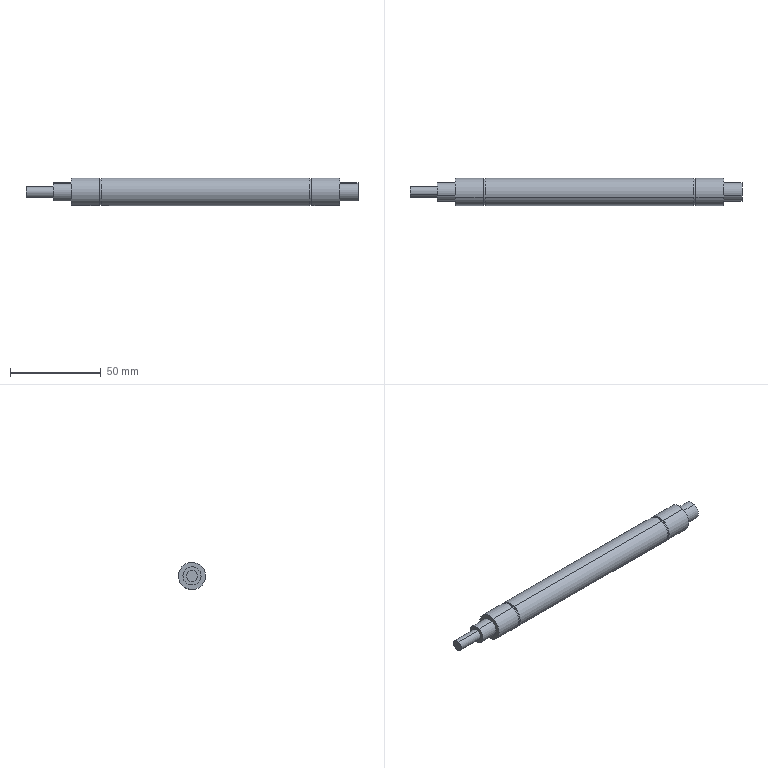Component | SolidWorks | GuideMechanism-1_RollerAxis01-1 | 1 solid | 31 faces | box 183 x 15 x 15 mm | volume 27756 mm3 | cylinder 19 | plane 12 | commonest cylinder face diameters 15 x6 10 x4 14 x4 5 x3 6 x2
build123d program:
from build123d import *

# Parameters (mm, degrees)
SKETCH1_W          = 183
SKETCH1_H          = 7.5
CUT_EXTRUDE1_START = -10
SKETCH2_R          = 7.5
SKETCH2_R_2        = 5
CUT_EXTRUDE1_DEPTH = 10
SKETCH3_R          = 7.5
SKETCH3_R_2        = 5
CUT_EXTRUDE2_DEPTH = 25
CUT_EXTRUDE3_DEPTH = 3
SKETCH6_R          = 5
SKETCH6_R_2        = 3
CUT_EXTRUDE4_DEPTH = 15
CUT_EXTRUDE5_START = -16.5
SKETCH7_R          = 7.5
SKETCH7_R_2        = 7
CUT_EXTRUDE5_DEPTH = 1.1
CUT_EXTRUDE6_START = -15.4
SKETCH8_R          = 7.5
SKETCH8_R_2        = 7
CUT_EXTRUDE6_DEPTH = 1.1


with BuildPart() as part:
    # Sketch1 → Revolve1 (revolve)
    with BuildSketch(Plane.XY, mode=Mode.PRIVATE) as revolve1_sk:
        with Locations((91.5, -3.75)):
            Rectangle(SKETCH1_W, SKETCH1_H)
    revolve(revolve1_sk.sketch.rotate(Axis((-439.507, 0, 0), (1, 0, 0)), 270), axis=Axis((-439.507, 0, 0), (1, 0, 0)))

    # Sketch2 → Cut-Extrude1 (cut)
    with BuildSketch(Plane.ZY.offset(CUT_EXTRUDE1_START)):
        Circle(SKETCH2_R)
        Circle(SKETCH2_R_2, mode=Mode.SUBTRACT)
    extrude(amount=CUT_EXTRUDE1_DEPTH, mode=Mode.SUBTRACT)

    # Sketch3 → Cut-Extrude2 (cut)
    with BuildSketch(Plane(origin=(183, 0, 0), x_dir=(0, 0, -1), z_dir=(1, 0, 0))):
        with Locations(Location((0, 0, 0), (0, 0, 180))):
            Circle(SKETCH3_R)
        with Locations(Location((0, 0, 0), (0, 0, 180))):
            Circle(SKETCH3_R_2, mode=Mode.SUBTRACT)
    extrude(amount=-CUT_EXTRUDE2_DEPTH, mode=Mode.SUBTRACT)

    # Sketch4 → Cut-Extrude3 (cut)
    with BuildSketch(Plane(origin=(0, 0, -7.5), x_dir=(-1, 0, 0), z_dir=(0, 0, -1))):
        with BuildLine():
            Line((-31.5, -2.5), (-51.5, -2.5))
            ThreePointArc((-51.5, -2.5), (-54, 0), (-51.5, 2.5))
            Line((-51.5, 2.5), (-31.5, 2.5))
            ThreePointArc((-31.5, 2.5), (-29, 0), (-31.5, -2.5))
        make_face()
    extrude(amount=-CUT_EXTRUDE3_DEPTH, mode=Mode.SUBTRACT)

    # Sketch6 → Cut-Extrude4 (cut)
    with BuildSketch(Plane(origin=(183, 0, 0), x_dir=(0, 0, -1), z_dir=(1, 0, 0))):
        Circle(SKETCH6_R)
        Circle(SKETCH6_R_2, mode=Mode.SUBTRACT)
    extrude(amount=-CUT_EXTRUDE4_DEPTH, mode=Mode.SUBTRACT)

    # Sketch7 → Cut-Extrude5 (cut)
    with BuildSketch(Plane.ZY.offset(-10).offset(CUT_EXTRUDE5_START)):
        Circle(SKETCH7_R)
        Circle(SKETCH7_R_2, mode=Mode.SUBTRACT)
    extrude(amount=CUT_EXTRUDE5_DEPTH, mode=Mode.SUBTRACT)

    # Sketch8 → Cut-Extrude6 (cut)
    with BuildSketch(Plane(origin=(158, 0, 0), x_dir=(0, 0, -1), z_dir=(1, 0, 0)).offset(CUT_EXTRUDE6_START)):
        with Locations(Location((0, 0, 0), (0, 0, 180))):
            Circle(SKETCH8_R)
        with Locations(Location((0, 0, 0), (0, 0, 180))):
            Circle(SKETCH8_R_2, mode=Mode.SUBTRACT)
    extrude(amount=-CUT_EXTRUDE6_DEPTH, mode=Mode.SUBTRACT)


solid = part.part

# Placed as in the assembly
solid = solid.moved(Location((-355.272, -352.564, 1209.912), (21.773, 0, 180)))
STEP:
#1=COLOUR_RGB('',0.7922,0.8196,0.9333);
#2=FILL_AREA_STYLE_COLOUR('',#1);
#3=FILL_AREA_STYLE('',(#2));
#4=SURFACE_STYLE_FILL_AREA(#3);
#5=SURFACE_SIDE_STYLE('',(#4));
#6=SURFACE_STYLE_USAGE(.BOTH.,#5);
#7=PRESENTATION_STYLE_ASSIGNMENT((#6));
#8=CARTESIAN_POINT('',(-20.208,-13.771,47.36));
#9=VERTEX_POINT('',#8);
#10=CARTESIAN_POINT('',(-20.208,-13.99,47.909));
#11=VERTEX_POINT('',#10);
#12=CARTESIAN_POINT('',(-20.208,-13.88,47.634));
#13=DIRECTION('',(-1.,-0.,-0.));
#14=DIRECTION('',(0.,0.3709,-0.9287));
#15=AXIS2_PLACEMENT_3D('',#12,#13,#14);
#16=CIRCLE('',#15,0.2953);
#17=EDGE_CURVE('',#9,#11,#16,.T.);
#18=ORIENTED_EDGE('',*,*,#17,.F.);
#19=CARTESIAN_POINT('',(-19.601,-13.771,47.36));
#20=VERTEX_POINT('',#19);
#21=CARTESIAN_POINT('',(3.316,-13.771,47.36));
#22=DIRECTION('',(1.,0.,0.));
#23=VECTOR('',#22,39.37);
#24=LINE('',#21,#23);
#25=EDGE_CURVE('',#9,#20,#24,.T.);
#26=ORIENTED_EDGE('',*,*,#25,.T.);
#27=CARTESIAN_POINT('',(-19.601,-13.99,47.909));
#28=VERTEX_POINT('',#27);
#29=CARTESIAN_POINT('',(-19.601,-13.88,47.634));
#30=DIRECTION('',(-1.,-0.,-0.));
#31=DIRECTION('',(0.,0.3709,-0.9287));
#32=AXIS2_PLACEMENT_3D('',#29,#30,#31);
#33=CIRCLE('',#32,0.2953);
#34=EDGE_CURVE('',#20,#28,#33,.T.);
#35=ORIENTED_EDGE('',*,*,#34,.T.);
#36=CARTESIAN_POINT('',(3.316,-13.99,47.909));
#37=DIRECTION('',(1.,0.,0.));
#38=VECTOR('',#37,39.37);
#39=LINE('',#36,#38);
#40=EDGE_CURVE('',#11,#28,#39,.T.);
#41=ORIENTED_EDGE('',*,*,#40,.F.);
#42=EDGE_LOOP('',(#18,#26,#35,#41));
#43=FACE_OUTER_BOUND('',#42,.T.);
#44=CARTESIAN_POINT('',(3.316,-13.88,47.634));
#45=DIRECTION('',(1.,0.,0.));
#46=DIRECTION('',(0.,-0.3709,0.9287));
#47=AXIS2_PLACEMENT_3D('',#44,#45,#46);
#48=CYLINDRICAL_SURFACE('',#47,0.2953);
#49=ADVANCED_FACE('',(#43),#48,.T.);
#50=CARTESIAN_POINT('',(-20.208,-13.807,47.452));
#51=VERTEX_POINT('',#50);
#52=CARTESIAN_POINT('',(-20.208,-13.953,47.817));
#53=VERTEX_POINT('',#52);
#54=CARTESIAN_POINT('',(-20.208,-13.88,47.634));
#55=DIRECTION('',(-1.,-0.,-0.));
#56=DIRECTION('',(0.,0.3709,-0.9287));
#57=AXIS2_PLACEMENT_3D('',#54,#55,#56);
#58=CIRCLE('',#57,0.1969);
#59=EDGE_CURVE('',#51,#53,#58,.T.);
#60=ORIENTED_EDGE('',*,*,#59,.T.);
#61=CARTESIAN_POINT('',(-20.601,-13.953,47.817));
#62=VERTEX_POINT('',#61);
#63=CARTESIAN_POINT('',(-20.208,-13.953,47.817));
#64=DIRECTION('',(-1.,-0.,-0.));
#65=VECTOR('',#64,39.37);
#66=LINE('',#63,#65);
#67=EDGE_CURVE('',#53,#62,#66,.T.);
#68=ORIENTED_EDGE('',*,*,#67,.T.);
#69=CARTESIAN_POINT('',(-20.601,-13.807,47.452));
#70=VERTEX_POINT('',#69);
#71=CARTESIAN_POINT('',(-20.601,-13.88,47.634));
#72=DIRECTION('',(-1.,-0.,-0.));
#73=DIRECTION('',(0.,0.3709,-0.9287));
#74=AXIS2_PLACEMENT_3D('',#71,#72,#73);
#75=CIRCLE('',#74,0.1969);
#76=EDGE_CURVE('',#70,#62,#75,.T.);
#77=ORIENTED_EDGE('',*,*,#76,.F.);
#78=CARTESIAN_POINT('',(-20.208,-13.807,47.452));
#79=DIRECTION('',(-1.,-0.,-0.));
#80=VECTOR('',#79,39.37);
#81=LINE('',#78,#80);
#82=EDGE_CURVE('',#51,#70,#81,.T.);
#83=ORIENTED_EDGE('',*,*,#82,.F.);
#84=EDGE_LOOP('',(#60,#68,#77,#83));
#85=FACE_OUTER_BOUND('',#84,.T.);
#86=CARTESIAN_POINT('',(-20.208,-13.88,47.634));
#87=DIRECTION('',(-1.,-0.,-0.));
#88=DIRECTION('',(0.,0.3709,-0.9287));
#89=AXIS2_PLACEMENT_3D('',#86,#87,#88);
#90=CYLINDRICAL_SURFACE('',#89,0.1969);
#91=ADVANCED_FACE('',(#85),#90,.T.);
#92=CARTESIAN_POINT('',(-20.601,-13.837,47.525));
#93=VERTEX_POINT('',#92);
#94=CARTESIAN_POINT('',(-20.601,-13.924,47.744));
#95=VERTEX_POINT('',#94);
#96=CARTESIAN_POINT('',(-20.601,-13.88,47.634));
#97=DIRECTION('',(-1.,-0.,-0.));
#98=DIRECTION('',(0.,0.3709,-0.9287));
#99=AXIS2_PLACEMENT_3D('',#96,#97,#98);
#100=CIRCLE('',#99,0.1181);
#101=EDGE_CURVE('',#93,#95,#100,.T.);
#102=ORIENTED_EDGE('',*,*,#101,.T.);
#103=CARTESIAN_POINT('',(-21.192,-13.924,47.744));
#104=VERTEX_POINT('',#103);
#105=CARTESIAN_POINT('',(-20.601,-13.924,47.744));
#106=DIRECTION('',(-1.,-0.,-0.));
#107=VECTOR('',#106,39.37);
#108=LINE('',#105,#107);
#109=EDGE_CURVE('',#95,#104,#108,.T.);
#110=ORIENTED_EDGE('',*,*,#109,.T.);
#111=CARTESIAN_POINT('',(-21.192,-13.837,47.525));
#112=VERTEX_POINT('',#111);
#113=CARTESIAN_POINT('',(-21.192,-13.88,47.634));
#114=DIRECTION('',(-1.,-0.,-0.));
#115=DIRECTION('',(0.,0.3709,-0.9287));
#116=AXIS2_PLACEMENT_3D('',#113,#114,#115);
#117=CIRCLE('',#116,0.1181);
#118=EDGE_CURVE('',#112,#104,#117,.T.);
#119=ORIENTED_EDGE('',*,*,#118,.F.);
#120=CARTESIAN_POINT('',(-20.601,-13.837,47.525));
#121=DIRECTION('',(-1.,-0.,-0.));
#122=VECTOR('',#121,39.37);
#123=LINE('',#120,#122);
#124=EDGE_CURVE('',#93,#112,#123,.T.);
#125=ORIENTED_EDGE('',*,*,#124,.F.);
#126=EDGE_LOOP('',(#102,#110,#119,#125));
#127=FACE_OUTER_BOUND('',#126,.T.);
#128=CARTESIAN_POINT('',(-20.601,-13.88,47.634));
#129=DIRECTION('',(-1.,-0.,-0.));
#130=DIRECTION('',(0.,0.3709,-0.9287));
#131=AXIS2_PLACEMENT_3D('',#128,#129,#130);
#132=CYLINDRICAL_SURFACE('',#131,0.1181);
#133=ADVANCED_FACE('',(#127),#132,.T.);
#134=CARTESIAN_POINT('',(-19.601,-13.778,47.378));
#135=VERTEX_POINT('',#134);
#136=CARTESIAN_POINT('',(-19.601,-13.983,47.89));
#137=VERTEX_POINT('',#136);
#138=CARTESIAN_POINT('',(-19.601,-13.88,47.634));
#139=DIRECTION('',(-1.,-0.,-0.));
#140=DIRECTION('',(0.,0.3709,-0.9287));
#141=AXIS2_PLACEMENT_3D('',#138,#139,#140);
#142=CIRCLE('',#141,0.2756);
#143=EDGE_CURVE('',#135,#137,#142,.T.);
#144=ORIENTED_EDGE('',*,*,#143,.F.);
#145=CARTESIAN_POINT('',(-19.558,-13.778,47.378));
#146=VERTEX_POINT('',#145);
#147=CARTESIAN_POINT('',(-19.601,-13.778,47.378));
#148=DIRECTION('',(1.,0.,0.));
#149=VECTOR('',#148,39.37);
#150=LINE('',#147,#149);
#151=EDGE_CURVE('',#135,#146,#150,.T.);
#152=ORIENTED_EDGE('',*,*,#151,.T.);
#153=CARTESIAN_POINT('',(-19.558,-13.983,47.89));
#154=VERTEX_POINT('',#153);
#155=CARTESIAN_POINT('',(-19.558,-13.88,47.634));
#156=DIRECTION('',(-1.,-0.,-0.));
#157=DIRECTION('',(0.,0.3709,-0.9287));
#158=AXIS2_PLACEMENT_3D('',#155,#156,#157);
#159=CIRCLE('',#158,0.2756);
#160=EDGE_CURVE('',#146,#154,#159,.T.);
#161=ORIENTED_EDGE('',*,*,#160,.T.);
#162=CARTESIAN_POINT('',(-19.601,-13.983,47.89));
#163=DIRECTION('',(1.,0.,0.));
#164=VECTOR('',#163,39.37);
#165=LINE('',#162,#164);
#166=EDGE_CURVE('',#137,#154,#165,.T.);
#167=ORIENTED_EDGE('',*,*,#166,.F.);
#168=EDGE_LOOP('',(#144,#152,#161,#167));
#169=FACE_OUTER_BOUND('',#168,.T.);
#170=CARTESIAN_POINT('',(-19.601,-13.88,47.634));
#171=DIRECTION('',(1.,0.,0.));
#172=DIRECTION('',(0.,-0.3709,0.9287));
#173=AXIS2_PLACEMENT_3D('',#170,#171,#172);
#174=CYLINDRICAL_SURFACE('',#173,0.2756);
#175=ADVANCED_FACE('',(#169),#174,.T.);
#176=CARTESIAN_POINT('',(-14.987,-13.99,47.909));
#177=VERTEX_POINT('',#176);
#178=CARTESIAN_POINT('',(-14.987,-13.771,47.36));
#179=VERTEX_POINT('',#178);
#180=CARTESIAN_POINT('',(-14.987,-13.88,47.634));
#181=DIRECTION('',(1.,0.,0.));
#182=DIRECTION('',(0.,-0.3709,0.9287));
#183=AXIS2_PLACEMENT_3D('',#180,#181,#182);
#184=CIRCLE('',#183,0.2953);
#185=EDGE_CURVE('',#177,#179,#184,.T.);
#186=ORIENTED_EDGE('',*,*,#185,.T.);
#187=CARTESIAN_POINT('',(-14.381,-13.771,47.36));
#188=VERTEX_POINT('',#187);
#189=CARTESIAN_POINT('',(3.316,-13.771,47.36));
#190=DIRECTION('',(1.,0.,0.));
#191=VECTOR('',#190,39.37);
#192=LINE('',#189,#191);
#193=EDGE_CURVE('',#179,#188,#192,.T.);
#194=ORIENTED_EDGE('',*,*,#193,.T.);
#195=CARTESIAN_POINT('',(-14.381,-13.99,47.909));
#196=VERTEX_POINT('',#195);
#197=CARTESIAN_POINT('',(-14.381,-13.88,47.634));
#198=DIRECTION('',(1.,0.,0.));
#199=DIRECTION('',(0.,-0.3709,0.9287));
#200=AXIS2_PLACEMENT_3D('',#197,#198,#199);
#201=CIRCLE('',#200,0.2953);
#202=EDGE_CURVE('',#196,#188,#201,.T.);
#203=ORIENTED_EDGE('',*,*,#202,.F.);
#204=CARTESIAN_POINT('',(3.316,-13.99,47.909));
#205=DIRECTION('',(1.,0.,0.));
#206=VECTOR('',#205,39.37);
#207=LINE('',#204,#206);
#208=EDGE_CURVE('',#177,#196,#207,.T.);
#209=ORIENTED_EDGE('',*,*,#208,.F.);
#210=EDGE_LOOP('',(#186,#194,#203,#209));
#211=FACE_OUTER_BOUND('',#210,.T.);
#212=CARTESIAN_POINT('',(3.316,-13.88,47.634));
#213=DIRECTION('',(1.,0.,0.));
#214=DIRECTION('',(0.,-0.3709,0.9287));
#215=AXIS2_PLACEMENT_3D('',#212,#213,#214);
#216=CYLINDRICAL_SURFACE('',#215,0.2953);
#217=ADVANCED_FACE('',(#211),#216,.T.);
#218=CARTESIAN_POINT('',(-14.381,-13.953,47.817));
#219=VERTEX_POINT('',#218);
#220=CARTESIAN_POINT('',(-14.381,-13.807,47.452));
#221=VERTEX_POINT('',#220);
#222=CARTESIAN_POINT('',(-14.381,-13.88,47.634));
#223=DIRECTION('',(1.,0.,0.));
#224=DIRECTION('',(0.,-0.3709,0.9287));
#225=AXIS2_PLACEMENT_3D('',#222,#223,#224);
#226=CIRCLE('',#225,0.1969);
#227=EDGE_CURVE('',#219,#221,#226,.T.);
#228=ORIENTED_EDGE('',*,*,#227,.T.);
#229=CARTESIAN_POINT('',(-13.987,-13.807,47.452));
#230=VERTEX_POINT('',#229);
#231=CARTESIAN_POINT('',(-14.381,-13.807,47.452));
#232=DIRECTION('',(1.,0.,0.));
#233=VECTOR('',#232,39.37);
#234=LINE('',#231,#233);
#235=EDGE_CURVE('',#221,#230,#234,.T.);
#236=ORIENTED_EDGE('',*,*,#235,.T.);
#237=CARTESIAN_POINT('',(-13.987,-13.953,47.817));
#238=VERTEX_POINT('',#237);
#239=CARTESIAN_POINT('',(-13.987,-13.88,47.634));
#240=DIRECTION('',(1.,0.,0.));
#241=DIRECTION('',(0.,-0.3709,0.9287));
#242=AXIS2_PLACEMENT_3D('',#239,#240,#241);
#243=CIRCLE('',#242,0.1969);
#244=EDGE_CURVE('',#238,#230,#243,.T.);
#245=ORIENTED_EDGE('',*,*,#244,.F.);
#246=CARTESIAN_POINT('',(-14.381,-13.953,47.817));
#247=DIRECTION('',(1.,0.,0.));
#248=VECTOR('',#247,39.37);
#249=LINE('',#246,#248);
#250=EDGE_CURVE('',#219,#238,#249,.T.);
#251=ORIENTED_EDGE('',*,*,#250,.F.);
#252=EDGE_LOOP('',(#228,#236,#245,#251));
#253=FACE_OUTER_BOUND('',#252,.T.);
#254=CARTESIAN_POINT('',(-14.381,-13.88,47.634));
#255=DIRECTION('',(1.,0.,0.));
#256=DIRECTION('',(0.,-0.3709,0.9287));
#257=AXIS2_PLACEMENT_3D('',#254,#255,#256);
#258=CYLINDRICAL_SURFACE('',#257,0.1969);
#259=ADVANCED_FACE('',(#253),#258,.T.);
#260=CARTESIAN_POINT('',(-14.987,-13.983,47.89));
#261=VERTEX_POINT('',#260);
#262=CARTESIAN_POINT('',(-14.987,-13.778,47.378));
#263=VERTEX_POINT('',#262);
#264=CARTESIAN_POINT('',(-14.987,-13.88,47.634));
#265=DIRECTION('',(1.,0.,0.));
#266=DIRECTION('',(0.,-0.3709,0.9287));
#267=AXIS2_PLACEMENT_3D('',#264,#265,#266);
#268=CIRCLE('',#267,0.2756);
#269=EDGE_CURVE('',#261,#263,#268,.T.);
#270=ORIENTED_EDGE('',*,*,#269,.F.);
#271=CARTESIAN_POINT('',(-15.03,-13.983,47.89));
#272=VERTEX_POINT('',#271);
#273=CARTESIAN_POINT('',(-14.987,-13.983,47.89));
#274=DIRECTION('',(-1.,-0.,-0.));
#275=VECTOR('',#274,39.37);
#276=LINE('',#273,#275);
#277=EDGE_CURVE('',#261,#272,#276,.T.);
#278=ORIENTED_EDGE('',*,*,#277,.T.);
#279=CARTESIAN_POINT('',(-15.03,-13.778,47.378));
#280=VERTEX_POINT('',#279);
#281=CARTESIAN_POINT('',(-15.03,-13.88,47.634));
#282=DIRECTION('',(1.,0.,0.));
#283=DIRECTION('',(0.,-0.3709,0.9287));
#284=AXIS2_PLACEMENT_3D('',#281,#282,#283);
#285=CIRCLE('',#284,0.2756);
#286=EDGE_CURVE('',#272,#280,#285,.T.);
#287=ORIENTED_EDGE('',*,*,#286,.T.);
#288=CARTESIAN_POINT('',(-14.987,-13.778,47.378));
#289=DIRECTION('',(-1.,-0.,-0.));
#290=VECTOR('',#289,39.37);
#291=LINE('',#288,#290);
#292=EDGE_CURVE('',#263,#280,#291,.T.);
#293=ORIENTED_EDGE('',*,*,#292,.F.);
#294=EDGE_LOOP('',(#270,#278,#287,#293));
#295=FACE_OUTER_BOUND('',#294,.T.);
#296=CARTESIAN_POINT('',(-14.987,-13.88,47.634));
#297=DIRECTION('',(-1.,-0.,-0.));
#298=DIRECTION('',(0.,0.3709,-0.9287));
#299=AXIS2_PLACEMENT_3D('',#296,#297,#298);
#300=CYLINDRICAL_SURFACE('',#299,0.2756);
#301=ADVANCED_FACE('',(#295),#300,.T.);
#302=CARTESIAN_POINT('',(-15.129,-13.815,47.47));
#303=VERTEX_POINT('',#302);
#304=CARTESIAN_POINT('',(-15.227,-13.906,47.433));
#305=VERTEX_POINT('',#304);
#306=CARTESIAN_POINT('',(-15.227,-13.815,47.47));
#307=DIRECTION('',(0.,0.3709,-0.9287));
#308=DIRECTION('',(1.,0.,0.));
#309=AXIS2_PLACEMENT_3D('',#306,#307,#308);
#310=CIRCLE('',#309,0.09843);
#311=EDGE_CURVE('',#303,#305,#310,.T.);
#312=ORIENTED_EDGE('',*,*,#311,.F.);
#313=CARTESIAN_POINT('',(-15.129,-13.771,47.36));
#314=VERTEX_POINT('',#313);
#315=CARTESIAN_POINT('',(-15.129,-13.815,47.47));
#316=DIRECTION('',(0.,0.3709,-0.9287));
#317=VECTOR('',#316,39.37);
#318=LINE('',#315,#317);
#319=EDGE_CURVE('',#303,#314,#318,.T.);
#320=ORIENTED_EDGE('',*,*,#319,.T.);
#321=CARTESIAN_POINT('',(-15.227,-13.869,47.339));
#322=VERTEX_POINT('',#321);
#323=CARTESIAN_POINT('',(-15.129,-13.771,47.36));
#324=CARTESIAN_POINT('',(-15.129,-13.777,47.358));
#325=CARTESIAN_POINT('',(-15.129,-13.783,47.355));
#326=CARTESIAN_POINT('',(-15.132,-13.795,47.352));
#327=CARTESIAN_POINT('',(-15.134,-13.801,47.35));
#328=CARTESIAN_POINT('',(-15.139,-13.813,47.347));
#329=CARTESIAN_POINT('',(-15.142,-13.818,47.346));
#330=CARTESIAN_POINT('',(-15.149,-13.829,47.344));
#331=CARTESIAN_POINT('',(-15.153,-13.834,47.343));
#332=CARTESIAN_POINT('',(-15.162,-13.843,47.341));
#333=CARTESIAN_POINT('',(-15.167,-13.847,47.341));
#334=CARTESIAN_POINT('',(-15.178,-13.855,47.34));
#335=CARTESIAN_POINT('',(-15.183,-13.858,47.34));
#336=CARTESIAN_POINT('',(-15.195,-13.863,47.34));
#337=CARTESIAN_POINT('',(-15.201,-13.865,47.339));
#338=CARTESIAN_POINT('',(-15.214,-13.868,47.339));
#339=CARTESIAN_POINT('',(-15.221,-13.869,47.339));
#340=CARTESIAN_POINT('',(-15.227,-13.869,47.339));
#341=B_SPLINE_CURVE_WITH_KNOTS('',3,(#323,#324,#325,#326,#327,#328,#329,#330,#331,#332,#333,#334,#335,#336,#337,#338,#339,#340),.UNSPECIFIED.,.F.,.F.,(4,2,2,2,2,2,2,2,4),(0.003937,0.004429,0.004921,0.005412,0.005904,0.006395,0.006887,0.007378,0.00787),.UNSPECIFIED.);
#342=EDGE_CURVE('',#314,#322,#341,.T.);
#343=ORIENTED_EDGE('',*,*,#342,.T.);
#344=CARTESIAN_POINT('',(-15.227,-13.906,47.433));
#345=DIRECTION('',(0.,0.3709,-0.9287));
#346=VECTOR('',#345,39.37);
#347=LINE('',#344,#346);
#348=EDGE_CURVE('',#305,#322,#347,.T.);
#349=ORIENTED_EDGE('',*,*,#348,.F.);
#350=EDGE_LOOP('',(#312,#320,#343,#349));
#351=FACE_OUTER_BOUND('',#350,.T.);
#352=CARTESIAN_POINT('',(-15.227,-13.815,47.47));
#353=DIRECTION('',(0.,0.3709,-0.9287));
#354=DIRECTION('',(1.,0.,0.));
#355=AXIS2_PLACEMENT_3D('',#352,#353,#354);
#356=CYLINDRICAL_SURFACE('',#355,0.09843);
#357=ADVANCED_FACE('',(#351),#356,.F.);
#358=CARTESIAN_POINT('',(-19.558,-13.771,47.36));
#359=VERTEX_POINT('',#358);
#360=CARTESIAN_POINT('',(-19.558,-13.99,47.909));
#361=VERTEX_POINT('',#360);
#362=CARTESIAN_POINT('',(-19.558,-13.88,47.634));
#363=DIRECTION('',(-1.,-0.,-0.));
#364=DIRECTION('',(0.,0.3709,-0.9287));
#365=AXIS2_PLACEMENT_3D('',#362,#363,#364);
#366=CIRCLE('',#365,0.2953);
#367=EDGE_CURVE('',#359,#361,#366,.T.);
#368=ORIENTED_EDGE('',*,*,#367,.F.);
#369=CARTESIAN_POINT('',(-16.113,-13.771,47.36));
#370=VERTEX_POINT('',#369);
#371=CARTESIAN_POINT('',(3.316,-13.771,47.36));
#372=DIRECTION('',(1.,0.,0.));
#373=VECTOR('',#372,39.37);
#374=LINE('',#371,#373);
#375=EDGE_CURVE('',#359,#370,#374,.T.);
#376=ORIENTED_EDGE('',*,*,#375,.T.);
#377=CARTESIAN_POINT('',(-16.015,-13.869,47.339));
#378=VERTEX_POINT('',#377);
#379=CARTESIAN_POINT('',(-16.015,-13.869,47.339));
#380=CARTESIAN_POINT('',(-16.021,-13.869,47.339));
#381=CARTESIAN_POINT('',(-16.028,-13.868,47.339));
#382=CARTESIAN_POINT('',(-16.04,-13.865,47.339));
#383=CARTESIAN_POINT('',(-16.047,-13.863,47.34));
#384=CARTESIAN_POINT('',(-16.058,-13.858,47.34));
#385=CARTESIAN_POINT('',(-16.064,-13.855,47.34));
#386=CARTESIAN_POINT('',(-16.075,-13.847,47.341));
#387=CARTESIAN_POINT('',(-16.08,-13.843,47.341));
#388=CARTESIAN_POINT('',(-16.093,-13.829,47.343));
#389=CARTESIAN_POINT('',(-16.101,-13.819,47.345));
#390=CARTESIAN_POINT('',(-16.108,-13.801,47.35));
#391=CARTESIAN_POINT('',(-16.11,-13.795,47.352));
#392=CARTESIAN_POINT('',(-16.112,-13.783,47.356));
#393=CARTESIAN_POINT('',(-16.113,-13.777,47.358));
#394=CARTESIAN_POINT('',(-16.113,-13.771,47.36));
#395=B_SPLINE_CURVE_WITH_KNOTS('',3,(#379,#380,#381,#382,#383,#384,#385,#386,#387,#388,#389,#390,#391,#392,#393,#394),.UNSPECIFIED.,.F.,.F.,(4,2,2,2,2,2,2,4),(0.,0.0004922,0.0009844,0.001477,0.001969,0.002953,0.003445,0.003937),.UNSPECIFIED.);
#396=EDGE_CURVE('',#378,#370,#395,.T.);
#397=ORIENTED_EDGE('',*,*,#396,.F.);
#398=CARTESIAN_POINT('',(3.316,-13.869,47.339));
#399=DIRECTION('',(-1.,-0.,-0.));
#400=VECTOR('',#399,39.37);
#401=LINE('',#398,#400);
#402=EDGE_CURVE('',#322,#378,#401,.T.);
#403=ORIENTED_EDGE('',*,*,#402,.F.);
#404=ORIENTED_EDGE('',*,*,#342,.F.);
#405=CARTESIAN_POINT('',(-15.03,-13.771,47.36));
#406=VERTEX_POINT('',#405);
#407=CARTESIAN_POINT('',(3.316,-13.771,47.36));
#408=DIRECTION('',(1.,0.,0.));
#409=VECTOR('',#408,39.37);
#410=LINE('',#407,#409);
#411=EDGE_CURVE('',#314,#406,#410,.T.);
#412=ORIENTED_EDGE('',*,*,#411,.T.);
#413=CARTESIAN_POINT('',(-15.03,-13.99,47.909));
#414=VERTEX_POINT('',#413);
#415=CARTESIAN_POINT('',(-15.03,-13.88,47.634));
#416=DIRECTION('',(1.,0.,0.));
#417=DIRECTION('',(0.,-0.3709,0.9287));
#418=AXIS2_PLACEMENT_3D('',#415,#416,#417);
#419=CIRCLE('',#418,0.2953);
#420=EDGE_CURVE('',#414,#406,#419,.T.);
#421=ORIENTED_EDGE('',*,*,#420,.F.);
#422=CARTESIAN_POINT('',(3.316,-13.99,47.909));
#423=DIRECTION('',(1.,0.,0.));
#424=VECTOR('',#423,39.37);
#425=LINE('',#422,#424);
#426=EDGE_CURVE('',#361,#414,#425,.T.);
#427=ORIENTED_EDGE('',*,*,#426,.F.);
#428=EDGE_LOOP('',(#368,#376,#397,#403,#404,#412,#421,#427));
#429=FACE_OUTER_BOUND('',#428,.T.);
#430=CARTESIAN_POINT('',(3.316,-13.88,47.634));
#431=DIRECTION('',(1.,0.,0.));
#432=DIRECTION('',(0.,-0.3709,0.9287));
#433=AXIS2_PLACEMENT_3D('',#430,#431,#432);
#434=CYLINDRICAL_SURFACE('',#433,0.2953);
#435=ADVANCED_FACE('',(#429),#434,.T.);
#436=ORIENTED_EDGE('',*,*,#375,.F.);
#437=CARTESIAN_POINT('',(-19.558,-13.88,47.634));
#438=DIRECTION('',(-1.,-0.,-0.));
#439=DIRECTION('',(0.,0.3709,-0.9287));
#440=AXIS2_PLACEMENT_3D('',#437,#438,#439);
#441=CIRCLE('',#440,0.2953);
#442=EDGE_CURVE('',#361,#359,#441,.T.);
#443=ORIENTED_EDGE('',*,*,#442,.F.);
#444=ORIENTED_EDGE('',*,*,#426,.T.);
#445=CARTESIAN_POINT('',(-15.03,-13.88,47.634));
#446=DIRECTION('',(1.,0.,0.));
#447=DIRECTION('',(0.,-0.3709,0.9287));
#448=AXIS2_PLACEMENT_3D('',#445,#446,#447);
#449=CIRCLE('',#448,0.2953);
#450=EDGE_CURVE('',#406,#414,#449,.T.);
#451=ORIENTED_EDGE('',*,*,#450,.F.);
#452=ORIENTED_EDGE('',*,*,#411,.F.);
#453=CARTESIAN_POINT('',(-15.227,-13.686,47.412));
#454=VERTEX_POINT('',#453);
#455=CARTESIAN_POINT('',(-15.227,-13.686,47.412));
#456=CARTESIAN_POINT('',(-15.221,-13.686,47.412));
#457=CARTESIAN_POINT('',(-15.214,-13.686,47.412));
#458=CARTESIAN_POINT('',(-15.202,-13.688,47.41));
#459=CARTESIAN_POINT('',(-15.195,-13.69,47.409));
#460=CARTESIAN_POINT('',(-15.183,-13.694,47.405));
#461=CARTESIAN_POINT('',(-15.178,-13.696,47.403));
#462=CARTESIAN_POINT('',(-15.167,-13.702,47.399));
#463=CARTESIAN_POINT('',(-15.162,-13.706,47.396));
#464=CARTESIAN_POINT('',(-15.149,-13.717,47.388));
#465=CARTESIAN_POINT('',(-15.141,-13.726,47.382));
#466=CARTESIAN_POINT('',(-15.134,-13.742,47.373));
#467=CARTESIAN_POINT('',(-15.132,-13.748,47.371));
#468=CARTESIAN_POINT('',(-15.129,-13.759,47.365));
#469=CARTESIAN_POINT('',(-15.129,-13.765,47.363));
#470=CARTESIAN_POINT('',(-15.129,-13.771,47.36));
#471=B_SPLINE_CURVE_WITH_KNOTS('',3,(#455,#456,#457,#458,#459,#460,#461,#462,#463,#464,#465,#466,#467,#468,#469,#470),.UNSPECIFIED.,.F.,.F.,(4,2,2,2,2,2,2,4),(0.,0.0004922,0.0009844,0.001477,0.001969,0.002953,0.003445,0.003937),.UNSPECIFIED.);
#472=EDGE_CURVE('',#454,#314,#471,.T.);
#473=ORIENTED_EDGE('',*,*,#472,.F.);
#474=CARTESIAN_POINT('',(-16.015,-13.686,47.412));
#475=VERTEX_POINT('',#474);
#476=CARTESIAN_POINT('',(3.316,-13.686,47.412));
#477=DIRECTION('',(1.,0.,0.));
#478=VECTOR('',#477,39.37);
#479=LINE('',#476,#478);
#480=EDGE_CURVE('',#475,#454,#479,.T.);
#481=ORIENTED_EDGE('',*,*,#480,.F.);
#482=CARTESIAN_POINT('',(-16.113,-13.771,47.36));
#483=CARTESIAN_POINT('',(-16.113,-13.765,47.363));
#484=CARTESIAN_POINT('',(-16.112,-13.759,47.365));
#485=CARTESIAN_POINT('',(-16.11,-13.747,47.371));
#486=CARTESIAN_POINT('',(-16.108,-13.742,47.373));
#487=CARTESIAN_POINT('',(-16.103,-13.731,47.379));
#488=CARTESIAN_POINT('',(-16.1,-13.727,47.382));
#489=CARTESIAN_POINT('',(-16.093,-13.717,47.388));
#490=CARTESIAN_POINT('',(-16.089,-13.713,47.391));
#491=CARTESIAN_POINT('',(-16.08,-13.706,47.396));
#492=CARTESIAN_POINT('',(-16.075,-13.702,47.399));
#493=CARTESIAN_POINT('',(-16.064,-13.696,47.403));
#494=CARTESIAN_POINT('',(-16.058,-13.694,47.405));
#495=CARTESIAN_POINT('',(-16.047,-13.69,47.409));
#496=CARTESIAN_POINT('',(-16.04,-13.688,47.41));
#497=CARTESIAN_POINT('',(-16.028,-13.686,47.412));
#498=CARTESIAN_POINT('',(-16.021,-13.686,47.412));
#499=CARTESIAN_POINT('',(-16.015,-13.686,47.412));
#500=B_SPLINE_CURVE_WITH_KNOTS('',3,(#482,#483,#484,#485,#486,#487,#488,#489,#490,#491,#492,#493,#494,#495,#496,#497,#498,#499),.UNSPECIFIED.,.F.,.F.,(4,2,2,2,2,2,2,2,4),(0.003937,0.004429,0.004921,0.005412,0.005904,0.006395,0.006887,0.007378,0.00787),.UNSPECIFIED.);
#501=EDGE_CURVE('',#370,#475,#500,.T.);
#502=ORIENTED_EDGE('',*,*,#501,.F.);
#503=EDGE_LOOP('',(#436,#443,#444,#451,#452,#473,#481,#502));
#504=FACE_OUTER_BOUND('',#503,.T.);
#505=CARTESIAN_POINT('',(3.316,-13.88,47.634));
#506=DIRECTION('',(1.,0.,0.));
#507=DIRECTION('',(0.,-0.3709,0.9287));
#508=AXIS2_PLACEMENT_3D('',#505,#506,#507);
#509=CYLINDRICAL_SURFACE('',#508,0.2953);
#510=ADVANCED_FACE('',(#504),#509,.T.);
#511=ORIENTED_EDGE('',*,*,#319,.F.);
#512=CARTESIAN_POINT('',(-15.227,-13.723,47.506));
#513=VERTEX_POINT('',#512);
#514=CARTESIAN_POINT('',(-15.227,-13.815,47.47));
#515=DIRECTION('',(0.,0.3709,-0.9287));
#516=DIRECTION('',(1.,0.,0.));
#517=AXIS2_PLACEMENT_3D('',#514,#515,#516);
#518=CIRCLE('',#517,0.09843);
#519=EDGE_CURVE('',#513,#303,#518,.T.);
#520=ORIENTED_EDGE('',*,*,#519,.F.);
#521=CARTESIAN_POINT('',(-15.227,-13.723,47.506));
#522=DIRECTION('',(0.,0.3709,-0.9287));
#523=VECTOR('',#522,39.37);
#524=LINE('',#521,#523);
#525=EDGE_CURVE('',#513,#454,#524,.T.);
#526=ORIENTED_EDGE('',*,*,#525,.T.);
#527=ORIENTED_EDGE('',*,*,#472,.T.);
#528=EDGE_LOOP('',(#511,#520,#526,#527));
#529=FACE_OUTER_BOUND('',#528,.T.);
#530=CARTESIAN_POINT('',(-15.227,-13.815,47.47));
#531=DIRECTION('',(0.,0.3709,-0.9287));
#532=DIRECTION('',(1.,0.,0.));
#533=AXIS2_PLACEMENT_3D('',#530,#531,#532);
#534=CYLINDRICAL_SURFACE('',#533,0.09843);
#535=ADVANCED_FACE('',(#529),#534,.F.);
#536=ORIENTED_EDGE('',*,*,#480,.T.);
#537=ORIENTED_EDGE('',*,*,#525,.F.);
#538=CARTESIAN_POINT('',(-16.015,-13.723,47.506));
#539=VERTEX_POINT('',#538);
#540=CARTESIAN_POINT('',(-15.227,-13.723,47.506));
#541=DIRECTION('',(1.,-0.,-0.));
#542=VECTOR('',#541,39.37);
#543=LINE('',#540,#542);
#544=EDGE_CURVE('',#539,#513,#543,.T.);
#545=ORIENTED_EDGE('',*,*,#544,.F.);
#546=CARTESIAN_POINT('',(-16.015,-13.723,47.506));
#547=DIRECTION('',(0.,0.3709,-0.9287));
#548=VECTOR('',#547,39.37);
#549=LINE('',#546,#548);
#550=EDGE_CURVE('',#539,#475,#549,.T.);
#551=ORIENTED_EDGE('',*,*,#550,.T.);
#552=EDGE_LOOP('',(#536,#537,#545,#551));
#553=FACE_OUTER_BOUND('',#552,.T.);
#554=CARTESIAN_POINT('',(-15.227,-13.723,47.506));
#555=DIRECTION('',(0.,0.9287,0.3709));
#556=DIRECTION('',(-1.,0.,0.));
#557=AXIS2_PLACEMENT_3D('',#554,#555,#556);
#558=PLANE('',#557);
#559=ADVANCED_FACE('',(#553),#558,.F.);
#560=CARTESIAN_POINT('',(-16.015,-13.906,47.433));
#561=VERTEX_POINT('',#560);
#562=CARTESIAN_POINT('',(-16.015,-13.906,47.433));
#563=DIRECTION('',(0.,0.3709,-0.9287));
#564=VECTOR('',#563,39.37);
#565=LINE('',#562,#564);
#566=EDGE_CURVE('',#561,#378,#565,.T.);
#567=ORIENTED_EDGE('',*,*,#566,.T.);
#568=ORIENTED_EDGE('',*,*,#396,.T.);
#569=ORIENTED_EDGE('',*,*,#501,.T.);
#570=ORIENTED_EDGE('',*,*,#550,.F.);
#571=CARTESIAN_POINT('',(-16.015,-13.815,47.47));
#572=DIRECTION('',(0.,0.3709,-0.9287));
#573=DIRECTION('',(1.,0.,0.));
#574=AXIS2_PLACEMENT_3D('',#571,#572,#573);
#575=CIRCLE('',#574,0.09843);
#576=EDGE_CURVE('',#561,#539,#575,.T.);
#577=ORIENTED_EDGE('',*,*,#576,.F.);
#578=EDGE_LOOP('',(#567,#568,#569,#570,#577));
#579=FACE_OUTER_BOUND('',#578,.T.);
#580=CARTESIAN_POINT('',(-16.015,-13.815,47.47));
#581=DIRECTION('',(0.,0.3709,-0.9287));
#582=DIRECTION('',(1.,0.,0.));
#583=AXIS2_PLACEMENT_3D('',#580,#581,#582);
#584=CYLINDRICAL_SURFACE('',#583,0.09843);
#585=ADVANCED_FACE('',(#579),#584,.F.);
#586=ORIENTED_EDGE('',*,*,#402,.T.);
#587=ORIENTED_EDGE('',*,*,#566,.F.);
#588=CARTESIAN_POINT('',(-15.227,-13.906,47.433));
#589=DIRECTION('',(-1.,0.,-0.));
#590=VECTOR('',#589,39.37);
#591=LINE('',#588,#590);
#592=EDGE_CURVE('',#305,#561,#591,.T.);
#593=ORIENTED_EDGE('',*,*,#592,.F.);
#594=ORIENTED_EDGE('',*,*,#348,.T.);
#595=EDGE_LOOP('',(#586,#587,#593,#594));
#596=FACE_OUTER_BOUND('',#595,.T.);
#597=CARTESIAN_POINT('',(-15.227,-13.906,47.433));
#598=DIRECTION('',(-0.,-0.9287,-0.3709));
#599=DIRECTION('',(1.,-0.,0.));
#600=AXIS2_PLACEMENT_3D('',#597,#598,#599);
#601=PLANE('',#600);
#602=ADVANCED_FACE('',(#596),#601,.F.);
#603=ORIENTED_EDGE('',*,*,#519,.T.);
#604=ORIENTED_EDGE('',*,*,#311,.T.);
#605=ORIENTED_EDGE('',*,*,#592,.T.);
#606=ORIENTED_EDGE('',*,*,#576,.T.);
#607=ORIENTED_EDGE('',*,*,#544,.T.);
#608=EDGE_LOOP('',(#603,#604,#605,#606,#607));
#609=FACE_OUTER_BOUND('',#608,.T.);
#610=CARTESIAN_POINT('',(-15.227,-13.815,47.47));
#611=DIRECTION('',(0.,0.3709,-0.9287));
#612=DIRECTION('',(1.,0.,0.));
#613=AXIS2_PLACEMENT_3D('',#610,#611,#612);
#614=PLANE('',#613);
#615=ADVANCED_FACE('',(#609),#614,.T.);
#616=ORIENTED_EDGE('',*,*,#185,.F.);
#617=CARTESIAN_POINT('',(-14.987,-13.88,47.634));
#618=DIRECTION('',(1.,0.,0.));
#619=DIRECTION('',(0.,-0.3709,0.9287));
#620=AXIS2_PLACEMENT_3D('',#617,#618,#619);
#621=CIRCLE('',#620,0.2953);
#622=EDGE_CURVE('',#179,#177,#621,.T.);
#623=ORIENTED_EDGE('',*,*,#622,.F.);
#624=EDGE_LOOP('',(#616,#623));
#625=FACE_OUTER_BOUND('',#624,.T.);
#626=CARTESIAN_POINT('',(-14.987,-13.88,47.634));
#627=DIRECTION('',(1.,0.,0.));
#628=DIRECTION('',(0.,-0.3709,0.9287));
#629=AXIS2_PLACEMENT_3D('',#626,#627,#628);
#630=CIRCLE('',#629,0.2756);
#631=EDGE_CURVE('',#263,#261,#630,.T.);
#632=ORIENTED_EDGE('',*,*,#631,.T.);
#633=ORIENTED_EDGE('',*,*,#269,.T.);
#634=EDGE_LOOP('',(#632,#633));
#635=FACE_BOUND('',#634,.T.);
#636=CARTESIAN_POINT('',(-14.987,-13.88,47.634));
#637=DIRECTION('',(1.,0.,0.));
#638=DIRECTION('',(-0.,-0.3709,0.9287));
#639=AXIS2_PLACEMENT_3D('',#636,#637,#638);
#640=PLANE('',#639);
#641=ADVANCED_FACE('',(#625,#635),#640,.F.);
#642=ORIENTED_EDGE('',*,*,#420,.T.);
#643=ORIENTED_EDGE('',*,*,#450,.T.);
#644=EDGE_LOOP('',(#642,#643));
#645=FACE_OUTER_BOUND('',#644,.T.);
#646=CARTESIAN_POINT('',(-15.03,-13.88,47.634));
#647=DIRECTION('',(1.,0.,0.));
#648=DIRECTION('',(0.,-0.3709,0.9287));
#649=AXIS2_PLACEMENT_3D('',#646,#647,#648);
#650=CIRCLE('',#649,0.2756);
#651=EDGE_CURVE('',#280,#272,#650,.T.);
#652=ORIENTED_EDGE('',*,*,#651,.F.);
#653=ORIENTED_EDGE('',*,*,#286,.F.);
#654=EDGE_LOOP('',(#652,#653));
#655=FACE_BOUND('',#654,.T.);
#656=CARTESIAN_POINT('',(-15.03,-13.88,47.634));
#657=DIRECTION('',(1.,0.,0.));
#658=DIRECTION('',(-0.,-0.3709,0.9287));
#659=AXIS2_PLACEMENT_3D('',#656,#657,#658);
#660=PLANE('',#659);
#661=ADVANCED_FACE('',(#645,#655),#660,.T.);
#662=ORIENTED_EDGE('',*,*,#277,.F.);
#663=ORIENTED_EDGE('',*,*,#631,.F.);
#664=ORIENTED_EDGE('',*,*,#292,.T.);
#665=ORIENTED_EDGE('',*,*,#651,.T.);
#666=EDGE_LOOP('',(#662,#663,#664,#665));
#667=FACE_OUTER_BOUND('',#666,.T.);
#668=CARTESIAN_POINT('',(-14.987,-13.88,47.634));
#669=DIRECTION('',(-1.,-0.,-0.));
#670=DIRECTION('',(0.,0.3709,-0.9287));
#671=AXIS2_PLACEMENT_3D('',#668,#669,#670);
#672=CYLINDRICAL_SURFACE('',#671,0.2756);
#673=ADVANCED_FACE('',(#667),#672,.T.);
#674=ORIENTED_EDGE('',*,*,#244,.T.);
#675=CARTESIAN_POINT('',(-13.987,-13.88,47.634));
#676=DIRECTION('',(1.,0.,0.));
#677=DIRECTION('',(0.,-0.3709,0.9287));
#678=AXIS2_PLACEMENT_3D('',#675,#676,#677);
#679=CIRCLE('',#678,0.1969);
#680=EDGE_CURVE('',#230,#238,#679,.T.);
#681=ORIENTED_EDGE('',*,*,#680,.T.);
#682=EDGE_LOOP('',(#674,#681));
#683=FACE_OUTER_BOUND('',#682,.T.);
#684=CARTESIAN_POINT('',(-13.987,-13.88,47.634));
#685=DIRECTION('',(1.,0.,0.));
#686=DIRECTION('',(-0.,-0.3709,0.9287));
#687=AXIS2_PLACEMENT_3D('',#684,#685,#686);
#688=PLANE('',#687);
#689=ADVANCED_FACE('',(#683),#688,.T.);
#690=ORIENTED_EDGE('',*,*,#235,.F.);
#691=CARTESIAN_POINT('',(-14.381,-13.88,47.634));
#692=DIRECTION('',(1.,0.,0.));
#693=DIRECTION('',(0.,-0.3709,0.9287));
#694=AXIS2_PLACEMENT_3D('',#691,#692,#693);
#695=CIRCLE('',#694,0.1969);
#696=EDGE_CURVE('',#221,#219,#695,.T.);
#697=ORIENTED_EDGE('',*,*,#696,.T.);
#698=ORIENTED_EDGE('',*,*,#250,.T.);
#699=ORIENTED_EDGE('',*,*,#680,.F.);
#700=EDGE_LOOP('',(#690,#697,#698,#699));
#701=FACE_OUTER_BOUND('',#700,.T.);
#702=CARTESIAN_POINT('',(-14.381,-13.88,47.634));
#703=DIRECTION('',(1.,0.,0.));
#704=DIRECTION('',(0.,-0.3709,0.9287));
#705=AXIS2_PLACEMENT_3D('',#702,#703,#704);
#706=CYLINDRICAL_SURFACE('',#705,0.1969);
#707=ADVANCED_FACE('',(#701),#706,.T.);
#708=ORIENTED_EDGE('',*,*,#227,.F.);
#709=ORIENTED_EDGE('',*,*,#696,.F.);
#710=EDGE_LOOP('',(#708,#709));
#711=FACE_BOUND('',#710,.T.);
#712=ORIENTED_EDGE('',*,*,#202,.T.);
#713=CARTESIAN_POINT('',(-14.381,-13.88,47.634));
#714=DIRECTION('',(1.,0.,0.));
#715=DIRECTION('',(0.,-0.3709,0.9287));
#716=AXIS2_PLACEMENT_3D('',#713,#714,#715);
#717=CIRCLE('',#716,0.2953);
#718=EDGE_CURVE('',#188,#196,#717,.T.);
#719=ORIENTED_EDGE('',*,*,#718,.T.);
#720=EDGE_LOOP('',(#712,#719));
#721=FACE_OUTER_BOUND('',#720,.T.);
#722=CARTESIAN_POINT('',(-14.381,-13.88,47.634));
#723=DIRECTION('',(1.,0.,0.));
#724=DIRECTION('',(-0.,-0.3709,0.9287));
#725=AXIS2_PLACEMENT_3D('',#722,#723,#724);
#726=PLANE('',#725);
#727=ADVANCED_FACE('',(#711,#721),#726,.T.);
#728=ORIENTED_EDGE('',*,*,#193,.F.);
#729=ORIENTED_EDGE('',*,*,#622,.T.);
#730=ORIENTED_EDGE('',*,*,#208,.T.);
#731=ORIENTED_EDGE('',*,*,#718,.F.);
#732=EDGE_LOOP('',(#728,#729,#730,#731));
#733=FACE_OUTER_BOUND('',#732,.T.);
#734=CARTESIAN_POINT('',(3.316,-13.88,47.634));
#735=DIRECTION('',(1.,0.,0.));
#736=DIRECTION('',(0.,-0.3709,0.9287));
#737=AXIS2_PLACEMENT_3D('',#734,#735,#736);
#738=CYLINDRICAL_SURFACE('',#737,0.2953);
#739=ADVANCED_FACE('',(#733),#738,.T.);
#740=CARTESIAN_POINT('',(-19.601,-13.88,47.634));
#741=DIRECTION('',(-1.,-0.,-0.));
#742=DIRECTION('',(0.,0.3709,-0.9287));
#743=AXIS2_PLACEMENT_3D('',#740,#741,#742);
#744=CIRCLE('',#743,0.2953);
#745=EDGE_CURVE('',#28,#20,#744,.T.);
#746=ORIENTED_EDGE('',*,*,#745,.F.);
#747=ORIENTED_EDGE('',*,*,#34,.F.);
#748=EDGE_LOOP('',(#746,#747));
#749=FACE_OUTER_BOUND('',#748,.T.);
#750=CARTESIAN_POINT('',(-19.601,-13.88,47.634));
#751=DIRECTION('',(-1.,-0.,-0.));
#752=DIRECTION('',(0.,0.3709,-0.9287));
#753=AXIS2_PLACEMENT_3D('',#750,#751,#752);
#754=CIRCLE('',#753,0.2756);
#755=EDGE_CURVE('',#137,#135,#754,.T.);
#756=ORIENTED_EDGE('',*,*,#755,.T.);
#757=ORIENTED_EDGE('',*,*,#143,.T.);
#758=EDGE_LOOP('',(#756,#757));
#759=FACE_BOUND('',#758,.T.);
#760=CARTESIAN_POINT('',(-19.601,-13.88,47.634));
#761=DIRECTION('',(-1.,-0.,-0.));
#762=DIRECTION('',(0.,0.3709,-0.9287));
#763=AXIS2_PLACEMENT_3D('',#760,#761,#762);
#764=PLANE('',#763);
#765=ADVANCED_FACE('',(#749,#759),#764,.F.);
#766=ORIENTED_EDGE('',*,*,#442,.T.);
#767=ORIENTED_EDGE('',*,*,#367,.T.);
#768=EDGE_LOOP('',(#766,#767));
#769=FACE_OUTER_BOUND('',#768,.T.);
#770=CARTESIAN_POINT('',(-19.558,-13.88,47.634));
#771=DIRECTION('',(-1.,-0.,-0.));
#772=DIRECTION('',(0.,0.3709,-0.9287));
#773=AXIS2_PLACEMENT_3D('',#770,#771,#772);
#774=CIRCLE('',#773,0.2756);
#775=EDGE_CURVE('',#154,#146,#774,.T.);
#776=ORIENTED_EDGE('',*,*,#775,.F.);
#777=ORIENTED_EDGE('',*,*,#160,.F.);
#778=EDGE_LOOP('',(#776,#777));
#779=FACE_BOUND('',#778,.T.);
#780=CARTESIAN_POINT('',(-19.558,-13.88,47.634));
#781=DIRECTION('',(-1.,-0.,-0.));
#782=DIRECTION('',(0.,0.3709,-0.9287));
#783=AXIS2_PLACEMENT_3D('',#780,#781,#782);
#784=PLANE('',#783);
#785=ADVANCED_FACE('',(#769,#779),#784,.T.);
#786=ORIENTED_EDGE('',*,*,#151,.F.);
#787=ORIENTED_EDGE('',*,*,#755,.F.);
#788=ORIENTED_EDGE('',*,*,#166,.T.);
#789=ORIENTED_EDGE('',*,*,#775,.T.);
#790=EDGE_LOOP('',(#786,#787,#788,#789));
#791=FACE_OUTER_BOUND('',#790,.T.);
#792=CARTESIAN_POINT('',(-19.601,-13.88,47.634));
#793=DIRECTION('',(1.,0.,0.));
#794=DIRECTION('',(0.,-0.3709,0.9287));
#795=AXIS2_PLACEMENT_3D('',#792,#793,#794);
#796=CYLINDRICAL_SURFACE('',#795,0.2756);
#797=ADVANCED_FACE('',(#791),#796,.T.);
#798=ORIENTED_EDGE('',*,*,#118,.T.);
#799=CARTESIAN_POINT('',(-21.192,-13.88,47.634));
#800=DIRECTION('',(-1.,-0.,-0.));
#801=DIRECTION('',(0.,0.3709,-0.9287));
#802=AXIS2_PLACEMENT_3D('',#799,#800,#801);
#803=CIRCLE('',#802,0.1181);
#804=EDGE_CURVE('',#104,#112,#803,.T.);
#805=ORIENTED_EDGE('',*,*,#804,.T.);
#806=EDGE_LOOP('',(#798,#805));
#807=FACE_OUTER_BOUND('',#806,.T.);
#808=CARTESIAN_POINT('',(-21.192,-13.606,47.744));
#809=DIRECTION('',(-1.,-0.,-0.));
#810=DIRECTION('',(0.,0.3709,-0.9287));
#811=AXIS2_PLACEMENT_3D('',#808,#809,#810);
#812=PLANE('',#811);
#813=ADVANCED_FACE('',(#807),#812,.T.);
#814=ORIENTED_EDGE('',*,*,#109,.F.);
#815=CARTESIAN_POINT('',(-20.601,-13.88,47.634));
#816=DIRECTION('',(-1.,-0.,-0.));
#817=DIRECTION('',(0.,0.3709,-0.9287));
#818=AXIS2_PLACEMENT_3D('',#815,#816,#817);
#819=CIRCLE('',#818,0.1181);
#820=EDGE_CURVE('',#95,#93,#819,.T.);
#821=ORIENTED_EDGE('',*,*,#820,.T.);
#822=ORIENTED_EDGE('',*,*,#124,.T.);
#823=ORIENTED_EDGE('',*,*,#804,.F.);
#824=EDGE_LOOP('',(#814,#821,#822,#823));
#825=FACE_OUTER_BOUND('',#824,.T.);
#826=CARTESIAN_POINT('',(-20.601,-13.88,47.634));
#827=DIRECTION('',(-1.,-0.,-0.));
#828=DIRECTION('',(0.,0.3709,-0.9287));
#829=AXIS2_PLACEMENT_3D('',#826,#827,#828);
#830=CYLINDRICAL_SURFACE('',#829,0.1181);
#831=ADVANCED_FACE('',(#825),#830,.T.);
#832=ORIENTED_EDGE('',*,*,#101,.F.);
#833=ORIENTED_EDGE('',*,*,#820,.F.);
#834=EDGE_LOOP('',(#832,#833));
#835=FACE_BOUND('',#834,.T.);
#836=ORIENTED_EDGE('',*,*,#76,.T.);
#837=CARTESIAN_POINT('',(-20.601,-13.88,47.634));
#838=DIRECTION('',(-1.,-0.,-0.));
#839=DIRECTION('',(0.,0.3709,-0.9287));
#840=AXIS2_PLACEMENT_3D('',#837,#838,#839);
#841=CIRCLE('',#840,0.1969);
#842=EDGE_CURVE('',#62,#70,#841,.T.);
#843=ORIENTED_EDGE('',*,*,#842,.T.);
#844=EDGE_LOOP('',(#836,#843));
#845=FACE_OUTER_BOUND('',#844,.T.);
#846=CARTESIAN_POINT('',(-20.601,-13.88,47.634));
#847=DIRECTION('',(-1.,-0.,-0.));
#848=DIRECTION('',(0.,0.3709,-0.9287));
#849=AXIS2_PLACEMENT_3D('',#846,#847,#848);
#850=PLANE('',#849);
#851=ADVANCED_FACE('',(#835,#845),#850,.T.);
#852=ORIENTED_EDGE('',*,*,#67,.F.);
#853=CARTESIAN_POINT('',(-20.208,-13.88,47.634));
#854=DIRECTION('',(-1.,-0.,-0.));
#855=DIRECTION('',(0.,0.3709,-0.9287));
#856=AXIS2_PLACEMENT_3D('',#853,#854,#855);
#857=CIRCLE('',#856,0.1969);
#858=EDGE_CURVE('',#53,#51,#857,.T.);
#859=ORIENTED_EDGE('',*,*,#858,.T.);
#860=ORIENTED_EDGE('',*,*,#82,.T.);
#861=ORIENTED_EDGE('',*,*,#842,.F.);
#862=EDGE_LOOP('',(#852,#859,#860,#861));
#863=FACE_OUTER_BOUND('',#862,.T.);
#864=CARTESIAN_POINT('',(-20.208,-13.88,47.634));
#865=DIRECTION('',(-1.,-0.,-0.));
#866=DIRECTION('',(0.,0.3709,-0.9287));
#867=AXIS2_PLACEMENT_3D('',#864,#865,#866);
#868=CYLINDRICAL_SURFACE('',#867,0.1969);
#869=ADVANCED_FACE('',(#863),#868,.T.);
#870=ORIENTED_EDGE('',*,*,#59,.F.);
#871=ORIENTED_EDGE('',*,*,#858,.F.);
#872=EDGE_LOOP('',(#870,#871));
#873=FACE_BOUND('',#872,.T.);
#874=CARTESIAN_POINT('',(-20.208,-13.88,47.634));
#875=DIRECTION('',(-1.,-0.,-0.));
#876=DIRECTION('',(0.,0.3709,-0.9287));
#877=AXIS2_PLACEMENT_3D('',#874,#875,#876);
#878=CIRCLE('',#877,0.2953);
#879=EDGE_CURVE('',#11,#9,#878,.T.);
#880=ORIENTED_EDGE('',*,*,#879,.T.);
#881=ORIENTED_EDGE('',*,*,#17,.T.);
#882=EDGE_LOOP('',(#880,#881));
#883=FACE_OUTER_BOUND('',#882,.T.);
#884=CARTESIAN_POINT('',(-20.208,-13.88,47.634));
#885=DIRECTION('',(-1.,-0.,-0.));
#886=DIRECTION('',(0.,0.3709,-0.9287));
#887=AXIS2_PLACEMENT_3D('',#884,#885,#886);
#888=PLANE('',#887);
#889=ADVANCED_FACE('',(#873,#883),#888,.T.);
#890=ORIENTED_EDGE('',*,*,#25,.F.);
#891=ORIENTED_EDGE('',*,*,#879,.F.);
#892=ORIENTED_EDGE('',*,*,#40,.T.);
#893=ORIENTED_EDGE('',*,*,#745,.T.);
#894=EDGE_LOOP('',(#890,#891,#892,#893));
#895=FACE_OUTER_BOUND('',#894,.T.);
#896=CARTESIAN_POINT('',(3.316,-13.88,47.634));
#897=DIRECTION('',(1.,0.,0.));
#898=DIRECTION('',(0.,-0.3709,0.9287));
#899=AXIS2_PLACEMENT_3D('',#896,#897,#898);
#900=CYLINDRICAL_SURFACE('',#899,0.2953);
#901=ADVANCED_FACE('',(#895),#900,.T.);
#902=CLOSED_SHELL('',(#49,#91,#133,#175,#217,#259,#301,#357,#435,#510,#535,#559,#585,#602,#615,#641,#661,#673,#689,#707,#727,#739,#765,#785,#797,#813,#831,#851,#869,#889,#901));
#903=MANIFOLD_SOLID_BREP('',#902);
#904=STYLED_ITEM('',(#7),#903);
#905=(LENGTH_UNIT()NAMED_UNIT(*)SI_UNIT($,.METRE.));
#906=LENGTH_MEASURE_WITH_UNIT(LENGTH_MEASURE(0.0254),#905);
#907=DIMENSIONAL_EXPONENTS(1.,0.,0.,0.,0.,0.,0.);
#908=(CONVERSION_BASED_UNIT('',#906)LENGTH_UNIT()NAMED_UNIT(#907));
#909=UNCERTAINTY_MEASURE_WITH_UNIT(LENGTH_MEASURE(0.00001),#908,'','');
#910=(NAMED_UNIT(*)PLANE_ANGLE_UNIT()SI_UNIT($,.RADIAN.));
#911=(NAMED_UNIT(*)SI_UNIT($,.STERADIAN.)SOLID_ANGLE_UNIT());
#912=(GEOMETRIC_REPRESENTATION_CONTEXT(3)GLOBAL_UNCERTAINTY_ASSIGNED_CONTEXT((#909))GLOBAL_UNIT_ASSIGNED_CONTEXT((#908,#910,#911))REPRESENTATION_CONTEXT('',''));
#913=MECHANICAL_DESIGN_GEOMETRIC_PRESENTATION_REPRESENTATION('',(#904),#912);
#914=PRESENTATION_LAYER_ASSIGNMENT('','',(#904));
#915=CARTESIAN_POINT('',(0.,0.,0.));
#916=DIRECTION('',(0.,0.,1.));
#917=DIRECTION('',(1.,0.,0.));
#918=AXIS2_PLACEMENT_3D('',#915,#916,#917);
#919=(LENGTH_UNIT()NAMED_UNIT(*)SI_UNIT($,.METRE.));
#920=LENGTH_MEASURE_WITH_UNIT(LENGTH_MEASURE(0.0254),#919);
#921=DIMENSIONAL_EXPONENTS(1.,0.,0.,0.,0.,0.,0.);
#922=(CONVERSION_BASED_UNIT('',#920)LENGTH_UNIT()NAMED_UNIT(#921));
#923=UNCERTAINTY_MEASURE_WITH_UNIT(LENGTH_MEASURE(0.00001),#922,'','');
#924=(NAMED_UNIT(*)PLANE_ANGLE_UNIT()SI_UNIT($,.RADIAN.));
#925=(NAMED_UNIT(*)SI_UNIT($,.STERADIAN.)SOLID_ANGLE_UNIT());
#926=(GEOMETRIC_REPRESENTATION_CONTEXT(3)GLOBAL_UNCERTAINTY_ASSIGNED_CONTEXT((#923))GLOBAL_UNIT_ASSIGNED_CONTEXT((#922,#924,#925))REPRESENTATION_CONTEXT('',''));
#927=ADVANCED_BREP_SHAPE_REPRESENTATION('',(#903,#918),#926);